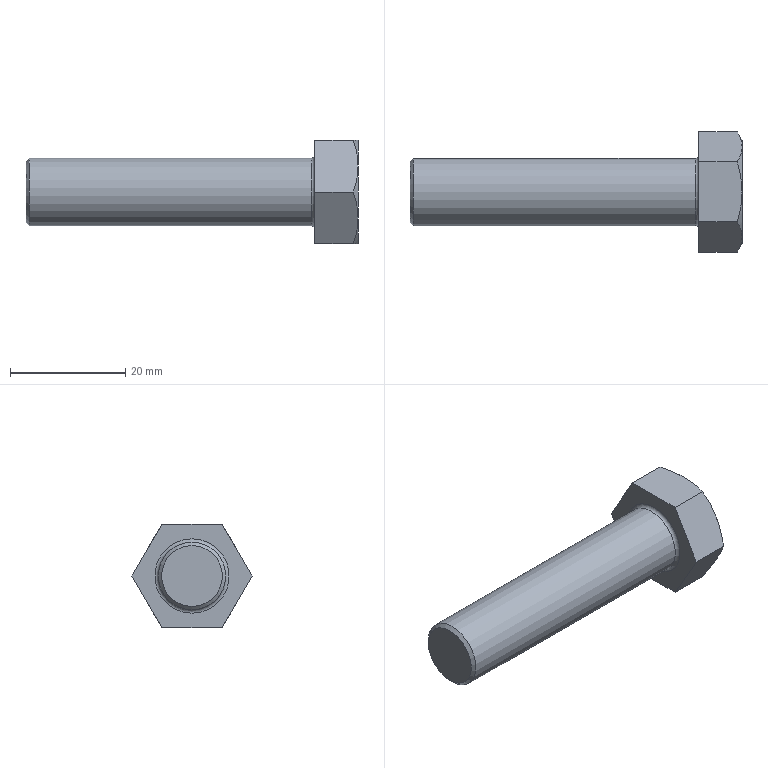Component | NX | GB-T5780-2000_M12X50 | 1 solid | 18 faces | volume 7471 mm3 | plane 9 | cone 7 | cylinder 1 | torus 1 | commonest cylinder face diameters 11.701 x1